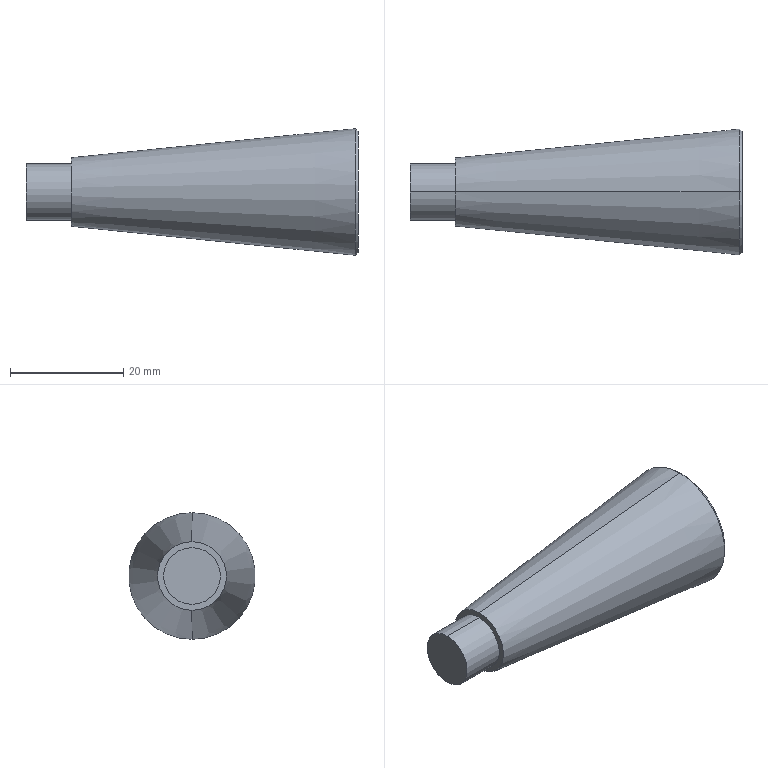Component | SolidWorks | Handle_2-1 | 1 solid | 9 faces | box 58.63 x 22.35 x 22.35 mm | volume 12854 mm3 | cone 4 | plane 3 | cylinder 2 | commonest cylinder face diameters 10 x2
build123d program:
from build123d import *

# Parameters (mm, degrees)
SKETCH1_R           = 5
BOSS_EXTRUDE1_DEPTH = 8
CHAMFER1_SIZE       = 0.5
CHAMFER1_SIZE2      = 0.456


with BuildPart() as part:
    # Sketch1 → Boss-Extrude1 (new body)
    with BuildSketch(Plane.XY):
        with Locations((15, 199.291)):
            Circle(SKETCH1_R)
    extrude(amount=-BOSS_EXTRUDE1_DEPTH)

    # Sketch2 → Revolve1 (revolve)
    with BuildSketch(Plane.ZY.offset(-15), mode=Mode.PRIVATE) as revolve1_sk:
        Polygon((0, 199.291), (0, 205.347), (50.631, 210.519), (50.631, 199.291), align=None)
    revolve(revolve1_sk.sketch.rotate(Axis((15, 199.291, 50.631), (0, 0, -1)), 90), axis=Axis((15, 199.291, 50.631), (0, 0, -1)))

    # Chamfer1
    chamfer1_edges = [part.edges().sort_by_distance(p)[0] for p in [
        (3.772, 199.291, 50.631),
    ]]
    chamfer1_side = [part.faces().sort_by_distance(p)[0] for p in [
        (6.358, 199.291, 25.316),
    ]]
    chamfer(chamfer1_edges, length=CHAMFER1_SIZE, length2=CHAMFER1_SIZE2, reference=chamfer1_side[0])


solid = part.part

# Placed as in the assembly
solid = solid.moved(Location((167.63, -7.481, 26.106), (0, 90, 0)))
STEP:
#1=COLOUR_RGB('',0.7922,0.8196,0.9333);
#2=FILL_AREA_STYLE_COLOUR('',#1);
#3=FILL_AREA_STYLE('',(#2));
#4=SURFACE_STYLE_FILL_AREA(#3);
#5=SURFACE_SIDE_STYLE('',(#4));
#6=SURFACE_STYLE_USAGE(.BOTH.,#5);
#7=PRESENTATION_STYLE_ASSIGNMENT((#6));
#8=CARTESIAN_POINT('',(8.593,7.552,0.01316));
#9=VERTEX_POINT('',#8);
#10=CARTESIAN_POINT('',(8.593,7.552,0.8613));
#11=VERTEX_POINT('',#10);
#12=CARTESIAN_POINT('',(8.593,7.552,0.4372));
#13=DIRECTION('',(1.,0.,0.));
#14=DIRECTION('',(0.,0.,-1.));
#15=AXIS2_PLACEMENT_3D('',#12,#13,#14);
#16=CIRCLE('',#15,0.4241);
#17=EDGE_CURVE('',#9,#11,#16,.T.);
#18=ORIENTED_EDGE('',*,*,#17,.F.);
#19=CARTESIAN_POINT('',(8.573,7.552,-0.002797));
#20=VERTEX_POINT('',#19);
#21=CARTESIAN_POINT('',(8.593,7.552,0.01316));
#22=DIRECTION('',(-0.7753,0.,-0.6316));
#23=VECTOR('',#22,39.37);
#24=LINE('',#21,#23);
#25=EDGE_CURVE('',#9,#20,#24,.T.);
#26=ORIENTED_EDGE('',*,*,#25,.T.);
#27=CARTESIAN_POINT('',(8.573,7.552,0.8773));
#28=VERTEX_POINT('',#27);
#29=CARTESIAN_POINT('',(8.573,7.552,0.4372));
#30=DIRECTION('',(-1.,-0.,-0.));
#31=DIRECTION('',(0.,0.,1.));
#32=AXIS2_PLACEMENT_3D('',#29,#30,#31);
#33=CIRCLE('',#32,0.44);
#34=EDGE_CURVE('',#28,#20,#33,.T.);
#35=ORIENTED_EDGE('',*,*,#34,.F.);
#36=CARTESIAN_POINT('',(8.593,7.552,0.8613));
#37=DIRECTION('',(-0.7753,-0.,0.6316));
#38=VECTOR('',#37,39.37);
#39=LINE('',#36,#38);
#40=EDGE_CURVE('',#11,#28,#39,.T.);
#41=ORIENTED_EDGE('',*,*,#40,.F.);
#42=EDGE_LOOP('',(#18,#26,#35,#41));
#43=FACE_OUTER_BOUND('',#42,.T.);
#44=CARTESIAN_POINT('',(8.593,7.552,0.4372));
#45=DIRECTION('',(-1.,-0.,-0.));
#46=DIRECTION('',(0.,0.,1.));
#47=AXIS2_PLACEMENT_3D('',#44,#45,#46);
#48=CONICAL_SURFACE('',#47,0.4241,0.6836);
#49=ADVANCED_FACE('',(#43),#48,.T.);
#50=CARTESIAN_POINT('',(6.6,7.552,0.1988));
#51=VERTEX_POINT('',#50);
#52=CARTESIAN_POINT('',(6.6,7.552,0.6757));
#53=VERTEX_POINT('',#52);
#54=CARTESIAN_POINT('',(6.6,7.552,0.4372));
#55=DIRECTION('',(1.,0.,0.));
#56=DIRECTION('',(0.,0.,-1.));
#57=AXIS2_PLACEMENT_3D('',#54,#55,#56);
#58=CIRCLE('',#57,0.2384);
#59=EDGE_CURVE('',#51,#53,#58,.T.);
#60=ORIENTED_EDGE('',*,*,#59,.T.);
#61=CARTESIAN_POINT('',(8.593,7.552,0.8793));
#62=DIRECTION('',(0.9948,0.,0.1016));
#63=VECTOR('',#62,39.37);
#64=LINE('',#61,#63);
#65=EDGE_CURVE('',#53,#28,#64,.T.);
#66=ORIENTED_EDGE('',*,*,#65,.T.);
#67=ORIENTED_EDGE('',*,*,#34,.T.);
#68=CARTESIAN_POINT('',(8.593,7.552,-0.004797));
#69=DIRECTION('',(0.9948,0.,-0.1016));
#70=VECTOR('',#69,39.37);
#71=LINE('',#68,#70);
#72=EDGE_CURVE('',#51,#20,#71,.T.);
#73=ORIENTED_EDGE('',*,*,#72,.F.);
#74=EDGE_LOOP('',(#60,#66,#67,#73));
#75=FACE_OUTER_BOUND('',#74,.T.);
#76=CARTESIAN_POINT('',(8.593,7.552,0.4372));
#77=DIRECTION('',(1.,0.,0.));
#78=DIRECTION('',(0.,0.,-1.));
#79=AXIS2_PLACEMENT_3D('',#76,#77,#78);
#80=CONICAL_SURFACE('',#79,0.442,0.1018);
#81=ADVANCED_FACE('',(#75),#80,.T.);
#82=CARTESIAN_POINT('',(6.285,7.552,0.2404));
#83=VERTEX_POINT('',#82);
#84=CARTESIAN_POINT('',(6.285,7.552,0.6341));
#85=VERTEX_POINT('',#84);
#86=CARTESIAN_POINT('',(6.285,7.552,0.4372));
#87=DIRECTION('',(1.,0.,0.));
#88=DIRECTION('',(0.,0.,-1.));
#89=AXIS2_PLACEMENT_3D('',#86,#87,#88);
#90=CIRCLE('',#89,0.1969);
#91=EDGE_CURVE('',#83,#85,#90,.T.);
#92=ORIENTED_EDGE('',*,*,#91,.T.);
#93=CARTESIAN_POINT('',(6.6,7.552,0.6341));
#94=VERTEX_POINT('',#93);
#95=CARTESIAN_POINT('',(6.285,7.552,0.6341));
#96=DIRECTION('',(1.,0.,0.));
#97=VECTOR('',#96,39.37);
#98=LINE('',#95,#97);
#99=EDGE_CURVE('',#85,#94,#98,.T.);
#100=ORIENTED_EDGE('',*,*,#99,.T.);
#101=CARTESIAN_POINT('',(6.6,7.552,0.2404));
#102=VERTEX_POINT('',#101);
#103=CARTESIAN_POINT('',(6.6,7.552,0.4372));
#104=DIRECTION('',(1.,0.,0.));
#105=DIRECTION('',(0.,0.,-1.));
#106=AXIS2_PLACEMENT_3D('',#103,#104,#105);
#107=CIRCLE('',#106,0.1969);
#108=EDGE_CURVE('',#102,#94,#107,.T.);
#109=ORIENTED_EDGE('',*,*,#108,.F.);
#110=CARTESIAN_POINT('',(6.285,7.552,0.2404));
#111=DIRECTION('',(1.,0.,0.));
#112=VECTOR('',#111,39.37);
#113=LINE('',#110,#112);
#114=EDGE_CURVE('',#83,#102,#113,.T.);
#115=ORIENTED_EDGE('',*,*,#114,.F.);
#116=EDGE_LOOP('',(#92,#100,#109,#115));
#117=FACE_OUTER_BOUND('',#116,.T.);
#118=CARTESIAN_POINT('',(6.285,7.552,0.4372));
#119=DIRECTION('',(1.,0.,0.));
#120=DIRECTION('',(0.,0.,-1.));
#121=AXIS2_PLACEMENT_3D('',#118,#119,#120);
#122=CYLINDRICAL_SURFACE('',#121,0.1969);
#123=ADVANCED_FACE('',(#117),#122,.T.);
#124=ORIENTED_EDGE('',*,*,#99,.F.);
#125=CARTESIAN_POINT('',(6.285,7.552,0.4372));
#126=DIRECTION('',(1.,0.,0.));
#127=DIRECTION('',(0.,0.,-1.));
#128=AXIS2_PLACEMENT_3D('',#125,#126,#127);
#129=CIRCLE('',#128,0.1969);
#130=EDGE_CURVE('',#85,#83,#129,.T.);
#131=ORIENTED_EDGE('',*,*,#130,.T.);
#132=ORIENTED_EDGE('',*,*,#114,.T.);
#133=CARTESIAN_POINT('',(6.6,7.552,0.4372));
#134=DIRECTION('',(1.,0.,0.));
#135=DIRECTION('',(0.,0.,-1.));
#136=AXIS2_PLACEMENT_3D('',#133,#134,#135);
#137=CIRCLE('',#136,0.1969);
#138=EDGE_CURVE('',#94,#102,#137,.T.);
#139=ORIENTED_EDGE('',*,*,#138,.F.);
#140=EDGE_LOOP('',(#124,#131,#132,#139));
#141=FACE_OUTER_BOUND('',#140,.T.);
#142=CARTESIAN_POINT('',(6.285,7.552,0.4372));
#143=DIRECTION('',(1.,0.,0.));
#144=DIRECTION('',(0.,0.,-1.));
#145=AXIS2_PLACEMENT_3D('',#142,#143,#144);
#146=CYLINDRICAL_SURFACE('',#145,0.1969);
#147=ADVANCED_FACE('',(#141),#146,.T.);
#148=ORIENTED_EDGE('',*,*,#91,.F.);
#149=ORIENTED_EDGE('',*,*,#130,.F.);
#150=EDGE_LOOP('',(#148,#149));
#151=FACE_OUTER_BOUND('',#150,.T.);
#152=CARTESIAN_POINT('',(6.285,7.552,0.4372));
#153=DIRECTION('',(1.,0.,0.));
#154=DIRECTION('',(0.,0.,-1.));
#155=AXIS2_PLACEMENT_3D('',#152,#153,#154);
#156=PLANE('',#155);
#157=ADVANCED_FACE('',(#151),#156,.F.);
#158=ORIENTED_EDGE('',*,*,#108,.T.);
#159=ORIENTED_EDGE('',*,*,#138,.T.);
#160=EDGE_LOOP('',(#158,#159));
#161=FACE_BOUND('',#160,.T.);
#162=ORIENTED_EDGE('',*,*,#59,.F.);
#163=CARTESIAN_POINT('',(6.6,7.552,0.4372));
#164=DIRECTION('',(1.,0.,0.));
#165=DIRECTION('',(0.,0.,-1.));
#166=AXIS2_PLACEMENT_3D('',#163,#164,#165);
#167=CIRCLE('',#166,0.2384);
#168=EDGE_CURVE('',#53,#51,#167,.T.);
#169=ORIENTED_EDGE('',*,*,#168,.F.);
#170=EDGE_LOOP('',(#162,#169));
#171=FACE_OUTER_BOUND('',#170,.T.);
#172=CARTESIAN_POINT('',(6.6,7.552,0.4372));
#173=DIRECTION('',(-1.,-0.,-0.));
#174=DIRECTION('',(-0.,-0.,1.));
#175=AXIS2_PLACEMENT_3D('',#172,#173,#174);
#176=PLANE('',#175);
#177=ADVANCED_FACE('',(#161,#171),#176,.T.);
#178=ORIENTED_EDGE('',*,*,#65,.F.);
#179=ORIENTED_EDGE('',*,*,#168,.T.);
#180=ORIENTED_EDGE('',*,*,#72,.T.);
#181=CARTESIAN_POINT('',(8.573,7.552,0.4372));
#182=DIRECTION('',(-1.,-0.,-0.));
#183=DIRECTION('',(0.,0.,1.));
#184=AXIS2_PLACEMENT_3D('',#181,#182,#183);
#185=CIRCLE('',#184,0.44);
#186=EDGE_CURVE('',#20,#28,#185,.T.);
#187=ORIENTED_EDGE('',*,*,#186,.T.);
#188=EDGE_LOOP('',(#178,#179,#180,#187));
#189=FACE_OUTER_BOUND('',#188,.T.);
#190=CARTESIAN_POINT('',(8.593,7.552,0.4372));
#191=DIRECTION('',(1.,0.,0.));
#192=DIRECTION('',(0.,0.,-1.));
#193=AXIS2_PLACEMENT_3D('',#190,#191,#192);
#194=CONICAL_SURFACE('',#193,0.442,0.1018);
#195=ADVANCED_FACE('',(#189),#194,.T.);
#196=CARTESIAN_POINT('',(8.593,7.552,0.4372));
#197=DIRECTION('',(1.,0.,0.));
#198=DIRECTION('',(0.,0.,-1.));
#199=AXIS2_PLACEMENT_3D('',#196,#197,#198);
#200=CIRCLE('',#199,0.4241);
#201=EDGE_CURVE('',#11,#9,#200,.T.);
#202=ORIENTED_EDGE('',*,*,#201,.T.);
#203=ORIENTED_EDGE('',*,*,#17,.T.);
#204=EDGE_LOOP('',(#202,#203));
#205=FACE_OUTER_BOUND('',#204,.T.);
#206=CARTESIAN_POINT('',(8.593,7.994,0.4372));
#207=DIRECTION('',(1.,0.,0.));
#208=DIRECTION('',(0.,0.,-1.));
#209=AXIS2_PLACEMENT_3D('',#206,#207,#208);
#210=PLANE('',#209);
#211=ADVANCED_FACE('',(#205),#210,.T.);
#212=ORIENTED_EDGE('',*,*,#25,.F.);
#213=ORIENTED_EDGE('',*,*,#201,.F.);
#214=ORIENTED_EDGE('',*,*,#40,.T.);
#215=ORIENTED_EDGE('',*,*,#186,.F.);
#216=EDGE_LOOP('',(#212,#213,#214,#215));
#217=FACE_OUTER_BOUND('',#216,.T.);
#218=CARTESIAN_POINT('',(8.593,7.552,0.4372));
#219=DIRECTION('',(-1.,-0.,-0.));
#220=DIRECTION('',(0.,0.,1.));
#221=AXIS2_PLACEMENT_3D('',#218,#219,#220);
#222=CONICAL_SURFACE('',#221,0.4241,0.6836);
#223=ADVANCED_FACE('',(#217),#222,.T.);
#224=CLOSED_SHELL('',(#49,#81,#123,#147,#157,#177,#195,#211,#223));
#225=MANIFOLD_SOLID_BREP('',#224);
#226=STYLED_ITEM('',(#7),#225);
#227=PRESENTATION_LAYER_ASSIGNMENT('','',(#226));
#228=CARTESIAN_POINT('',(0.,0.,0.));
#229=DIRECTION('',(0.,0.,1.));
#230=DIRECTION('',(1.,0.,0.));
#231=AXIS2_PLACEMENT_3D('',#228,#229,#230);
#232=(LENGTH_UNIT()NAMED_UNIT(*)SI_UNIT($,.METRE.));
#233=LENGTH_MEASURE_WITH_UNIT(LENGTH_MEASURE(0.0254),#232);
#234=DIMENSIONAL_EXPONENTS(1.,0.,0.,0.,0.,0.,0.);
#235=(CONVERSION_BASED_UNIT('',#233)LENGTH_UNIT()NAMED_UNIT(#234));
#236=UNCERTAINTY_MEASURE_WITH_UNIT(LENGTH_MEASURE(0.00001),#235,'','');
#237=(NAMED_UNIT(*)PLANE_ANGLE_UNIT()SI_UNIT($,.RADIAN.));
#238=(NAMED_UNIT(*)SI_UNIT($,.STERADIAN.)SOLID_ANGLE_UNIT());
#239=(GEOMETRIC_REPRESENTATION_CONTEXT(3)GLOBAL_UNCERTAINTY_ASSIGNED_CONTEXT((#236))GLOBAL_UNIT_ASSIGNED_CONTEXT((#235,#237,#238))REPRESENTATION_CONTEXT('',''));
#240=ADVANCED_BREP_SHAPE_REPRESENTATION('',(#225,#231),#239);
#241=(LENGTH_UNIT()NAMED_UNIT(*)SI_UNIT($,.METRE.));
#242=LENGTH_MEASURE_WITH_UNIT(LENGTH_MEASURE(0.0254),#241);
#243=DIMENSIONAL_EXPONENTS(1.,0.,0.,0.,0.,0.,0.);
#244=(CONVERSION_BASED_UNIT('',#242)LENGTH_UNIT()NAMED_UNIT(#243));
#245=UNCERTAINTY_MEASURE_WITH_UNIT(LENGTH_MEASURE(0.00001),#244,'','');
#246=(NAMED_UNIT(*)PLANE_ANGLE_UNIT()SI_UNIT($,.RADIAN.));
#247=(NAMED_UNIT(*)SI_UNIT($,.STERADIAN.)SOLID_ANGLE_UNIT());
#248=(GEOMETRIC_REPRESENTATION_CONTEXT(3)GLOBAL_UNCERTAINTY_ASSIGNED_CONTEXT((#245))GLOBAL_UNIT_ASSIGNED_CONTEXT((#244,#246,#247))REPRESENTATION_CONTEXT('',''));
#249=MECHANICAL_DESIGN_GEOMETRIC_PRESENTATION_REPRESENTATION('',(#226),#248);